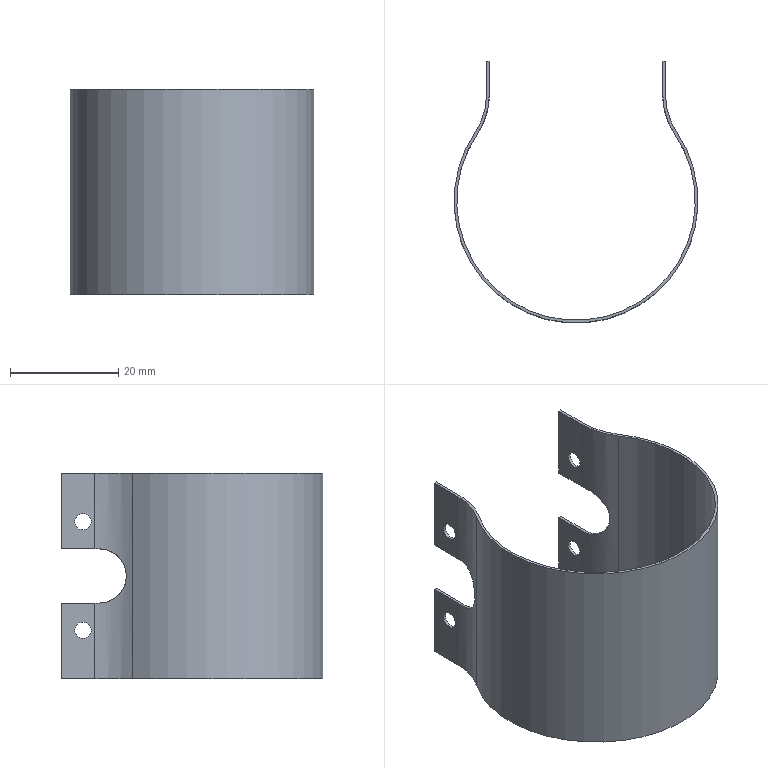Component | NX | OUTER_GUARD_PLATE | 1 solid | 30 faces | volume 2229 mm3 | plane 18 | cylinder 12 | commonest cylinder face diameters 3 x4 25 x2 26 x2 10 x2 45 x1 44 x1